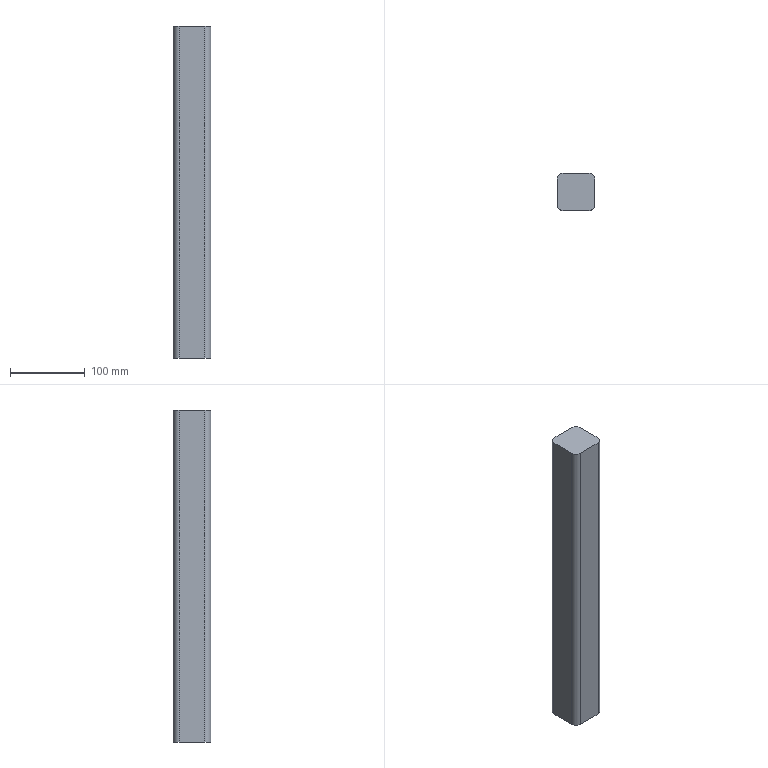Component | SolidWorks | AX00-100.1.1-1_AXFrame_A.1.1-1_AX50x50-1_square tube.1.1-5 | 1 solid | 20 faces | box 50 x 50 x 445 mm | volume 395413 mm3 | plane 12 | cylinder 8 | commonest cylinder face diameters 16 x4 6 x4 | material AISI 1035 Steel (SS)
build123d program:
from build123d import *

# Parameters (mm, degrees)
SKETCH1_W           = 50
SKETCH1_H           = 50
BOSS_EXTRUDE1_DEPTH = 222.5
FILLET3_R           = 8
SHELL1_T            = 5


with BuildPart() as part:
    # Sketch1 → Boss-Extrude1 (new, symmetric)
    with BuildSketch(Plane.XY):
        Rectangle(SKETCH1_W, SKETCH1_H)
    extrude(amount=BOSS_EXTRUDE1_DEPTH, both=True)

    # Fillet3
    fillet3_edges = [part.edges().sort_by_distance(p)[0] for p in [
        (25, -25, 0),
        (-25, -25, 0),
        (-25, 25, 0),
        (25, 25, 0),
    ]]
    fillet(fillet3_edges, radius=FILLET3_R)

    # Shell1 (no face opened: a closed hollow body)
    add(offset(amount=-SHELL1_T, mode=Mode.PRIVATE), mode=Mode.SUBTRACT)


solid = part.part

# Placed as in the assembly
solid = solid.moved(Location((1143.631, 1488.364, 0), (0, 0, 0)))